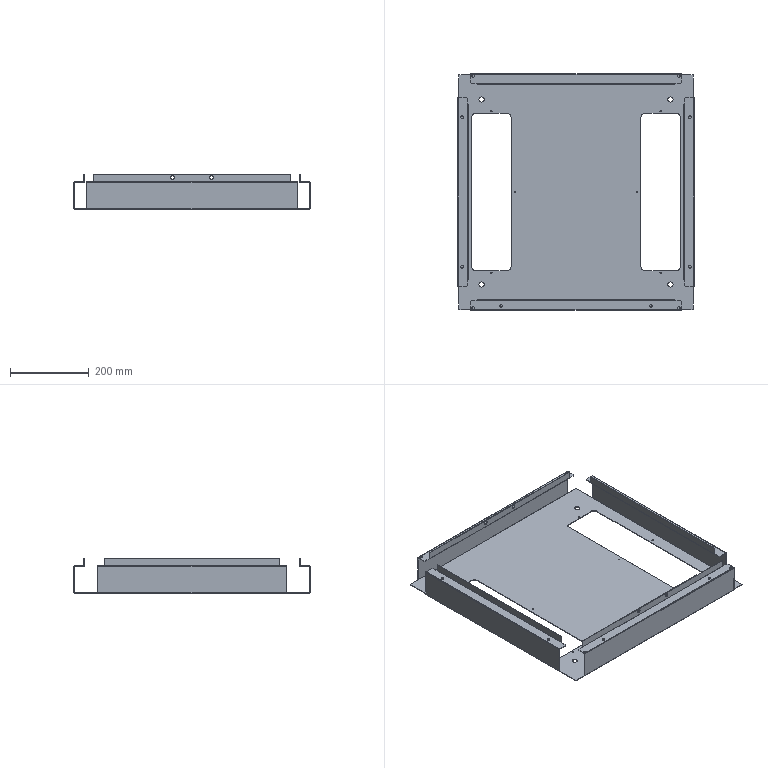Component | SolidWorks | Base-1 | 1 solid | 186 faces | volume 749064 mm3 | plane 110 | cylinder 76 | commonest cylinder face diameters 6.5 x20 3.3 x16 3 x12 9.2 x8 13 x8 20 x8 2 x4